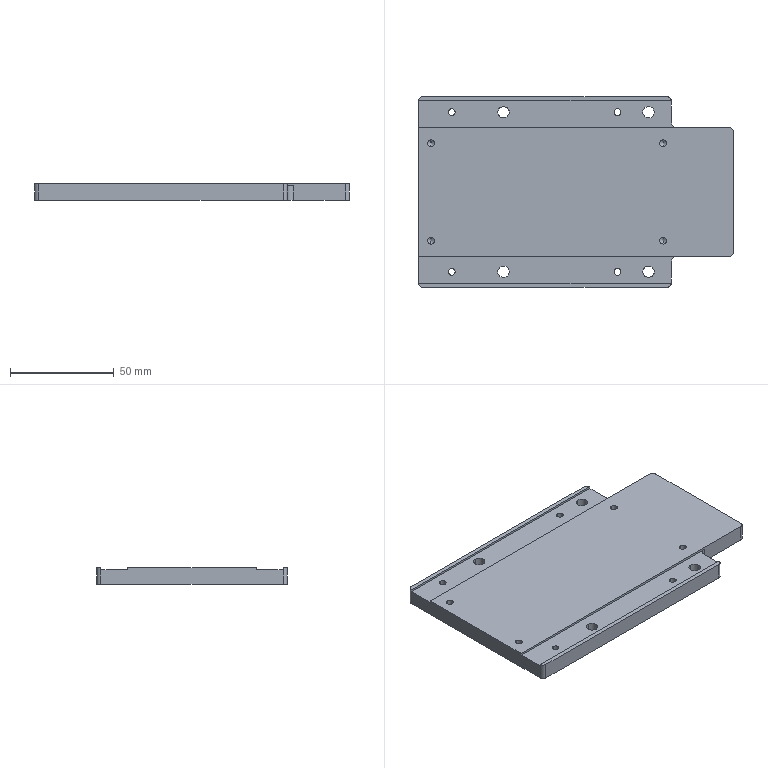CAM job | Mastercam | mm | 12 operations | part box 152 x 92 x 8
1. Facing | 24 - 63 平铣刀
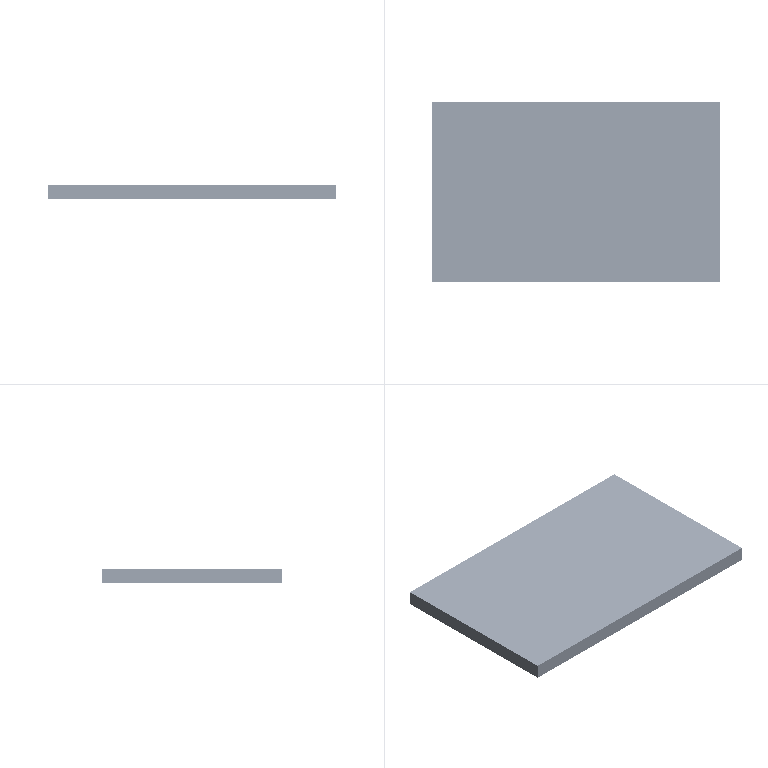2. 2D High Speed (2D Dynamic Mill) | 12 - 12 平铣刀
3. Contour (Ramp) | 12 - 12 平铣刀
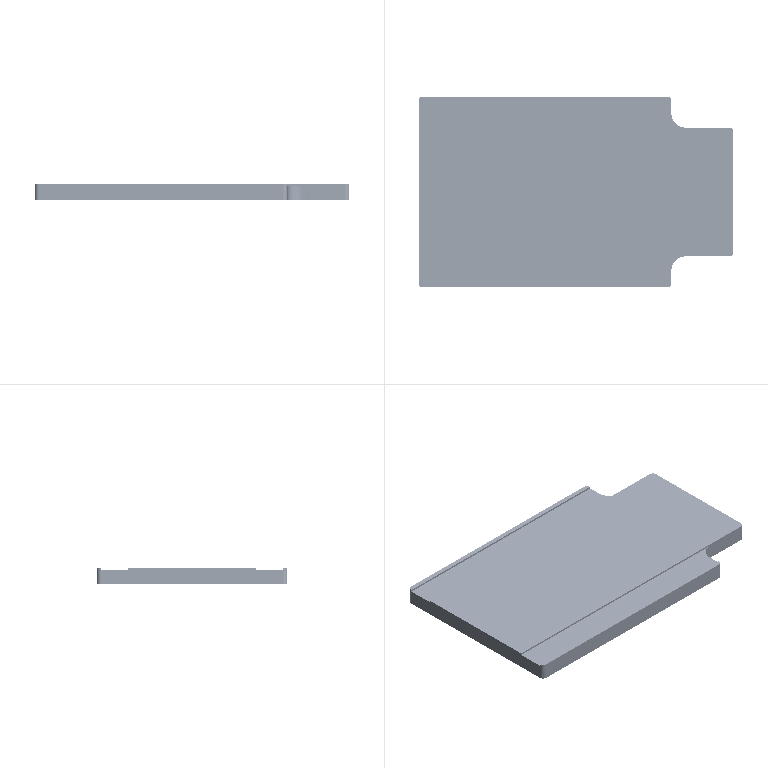4. Contour (Remachining) | 6 - 6 平铣刀
5. 2D High Speed (2D Area Mill) | 6 - 6 平铣刀
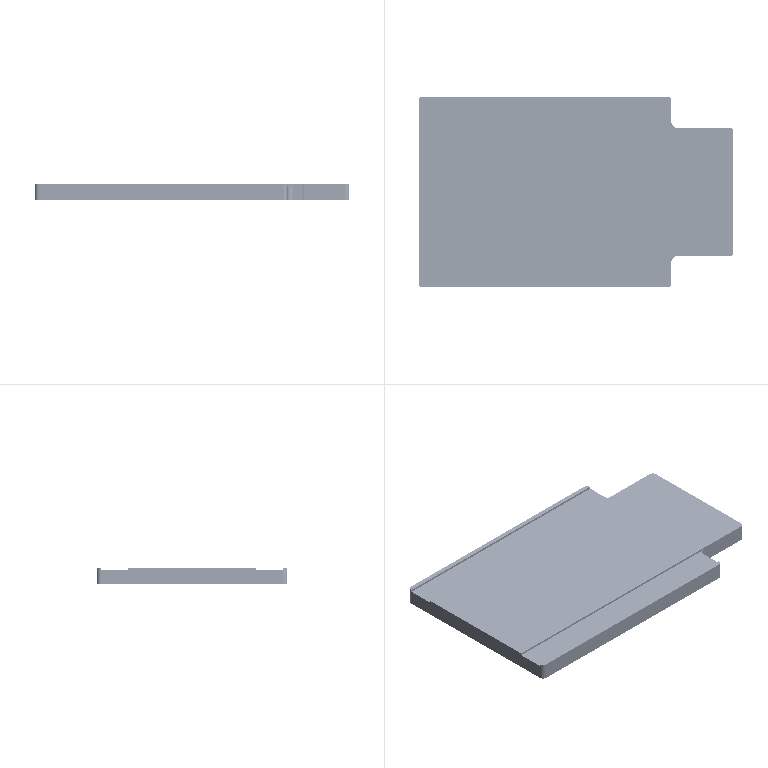6. Contour (2D) | 6 - 6 平铣刀
7. Contour (2D) | 6 - 6 平铣刀
8. Drill/Counterbore | 7 - 4 倒角刀
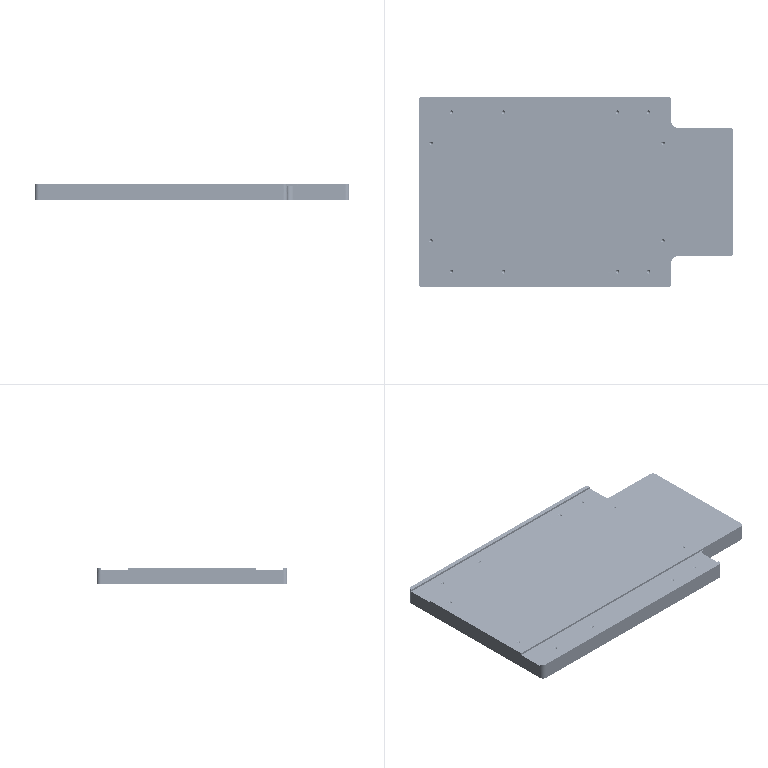9. Contour (2D chamfer) | 7 - 4 倒角刀
10. Facing | 12 - 12 平铣刀
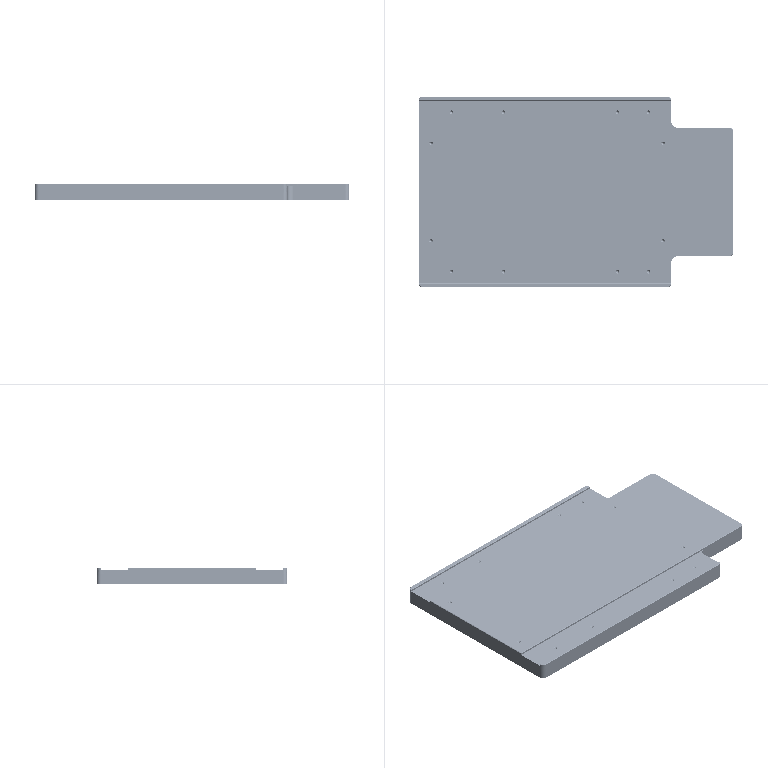11. Facing | 24 - 63 平铣刀
12. Contour (2D chamfer) | 7 - 4 倒角刀